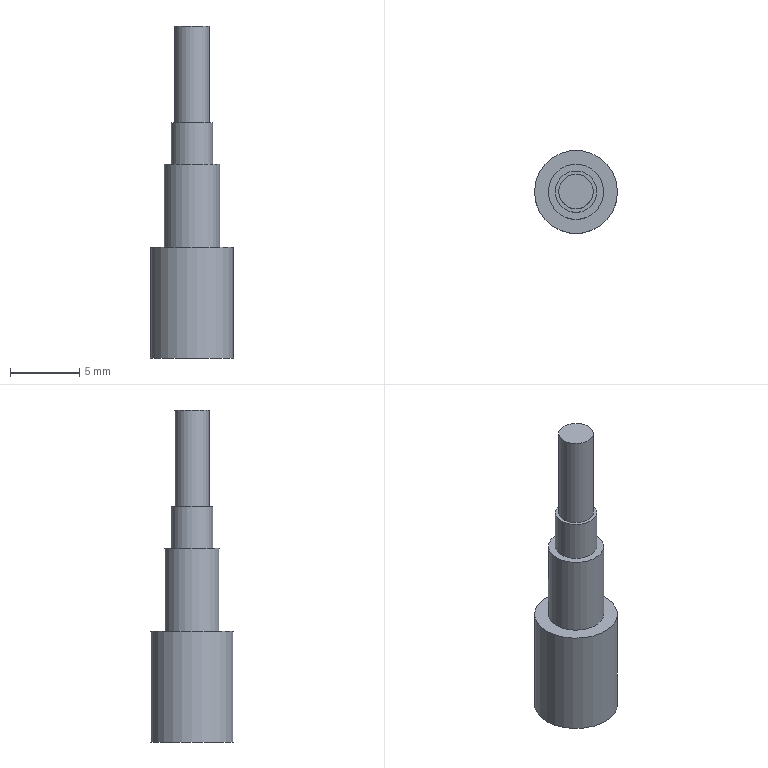Component | NX | VALVE_CORE | 1 solid | 9 faces | volume 357 mm3 | plane 5 | cylinder 4 | commonest cylinder face diameters 6 x1 4 x1 3 x1 2.5 x1